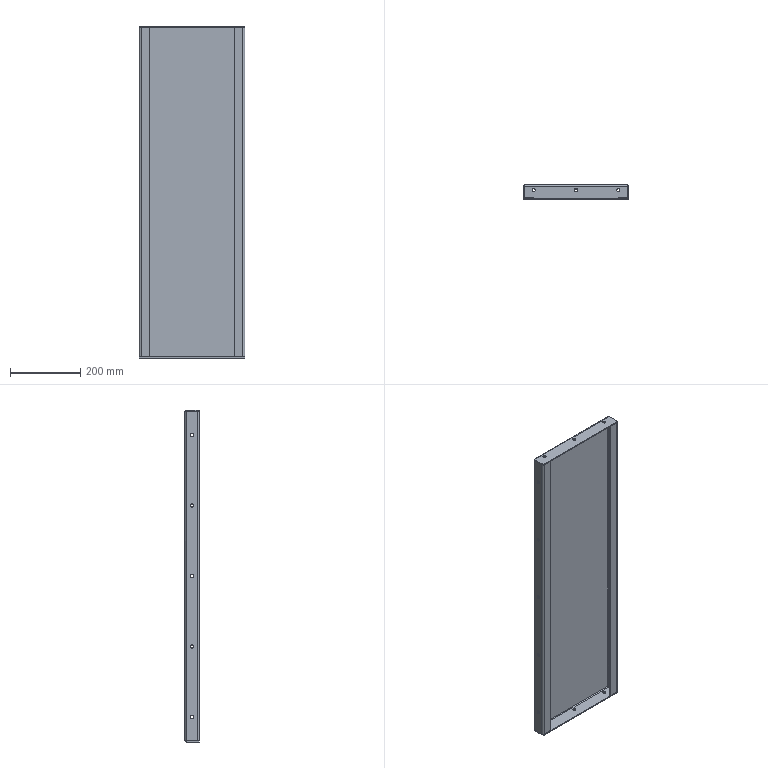Component | SolidWorks | ACBMountingPlateF5-1 | 1 solid | 86 faces | volume 1248184 mm3 | cylinder 44 | plane 34 | spline 8 | commonest cylinder face diameters 9 x32 5 x6 11 x6